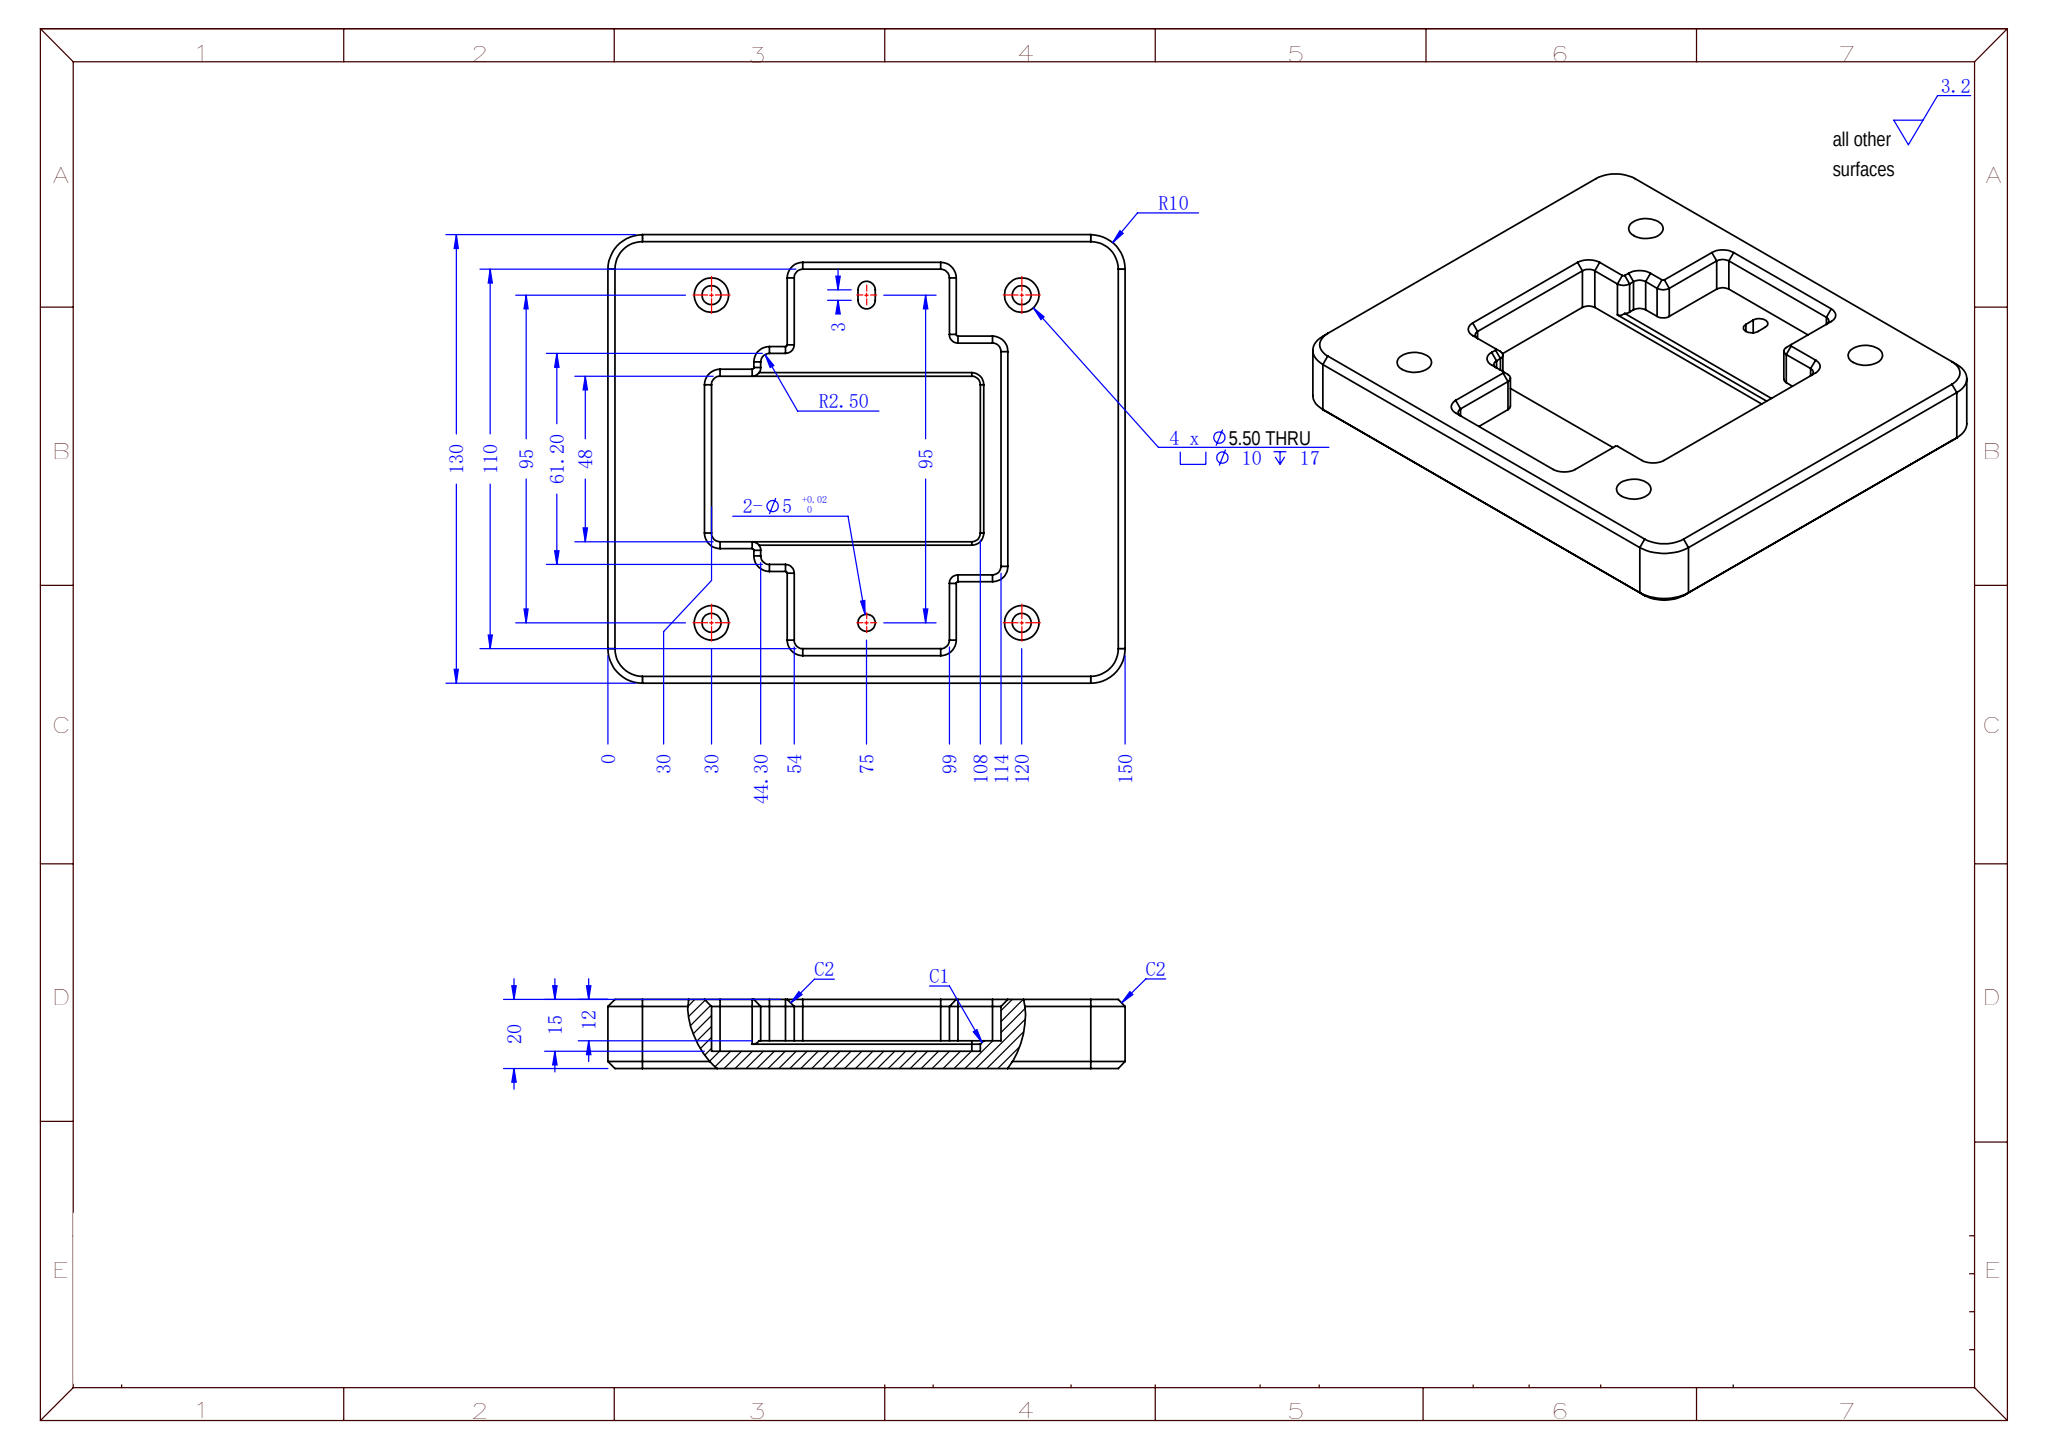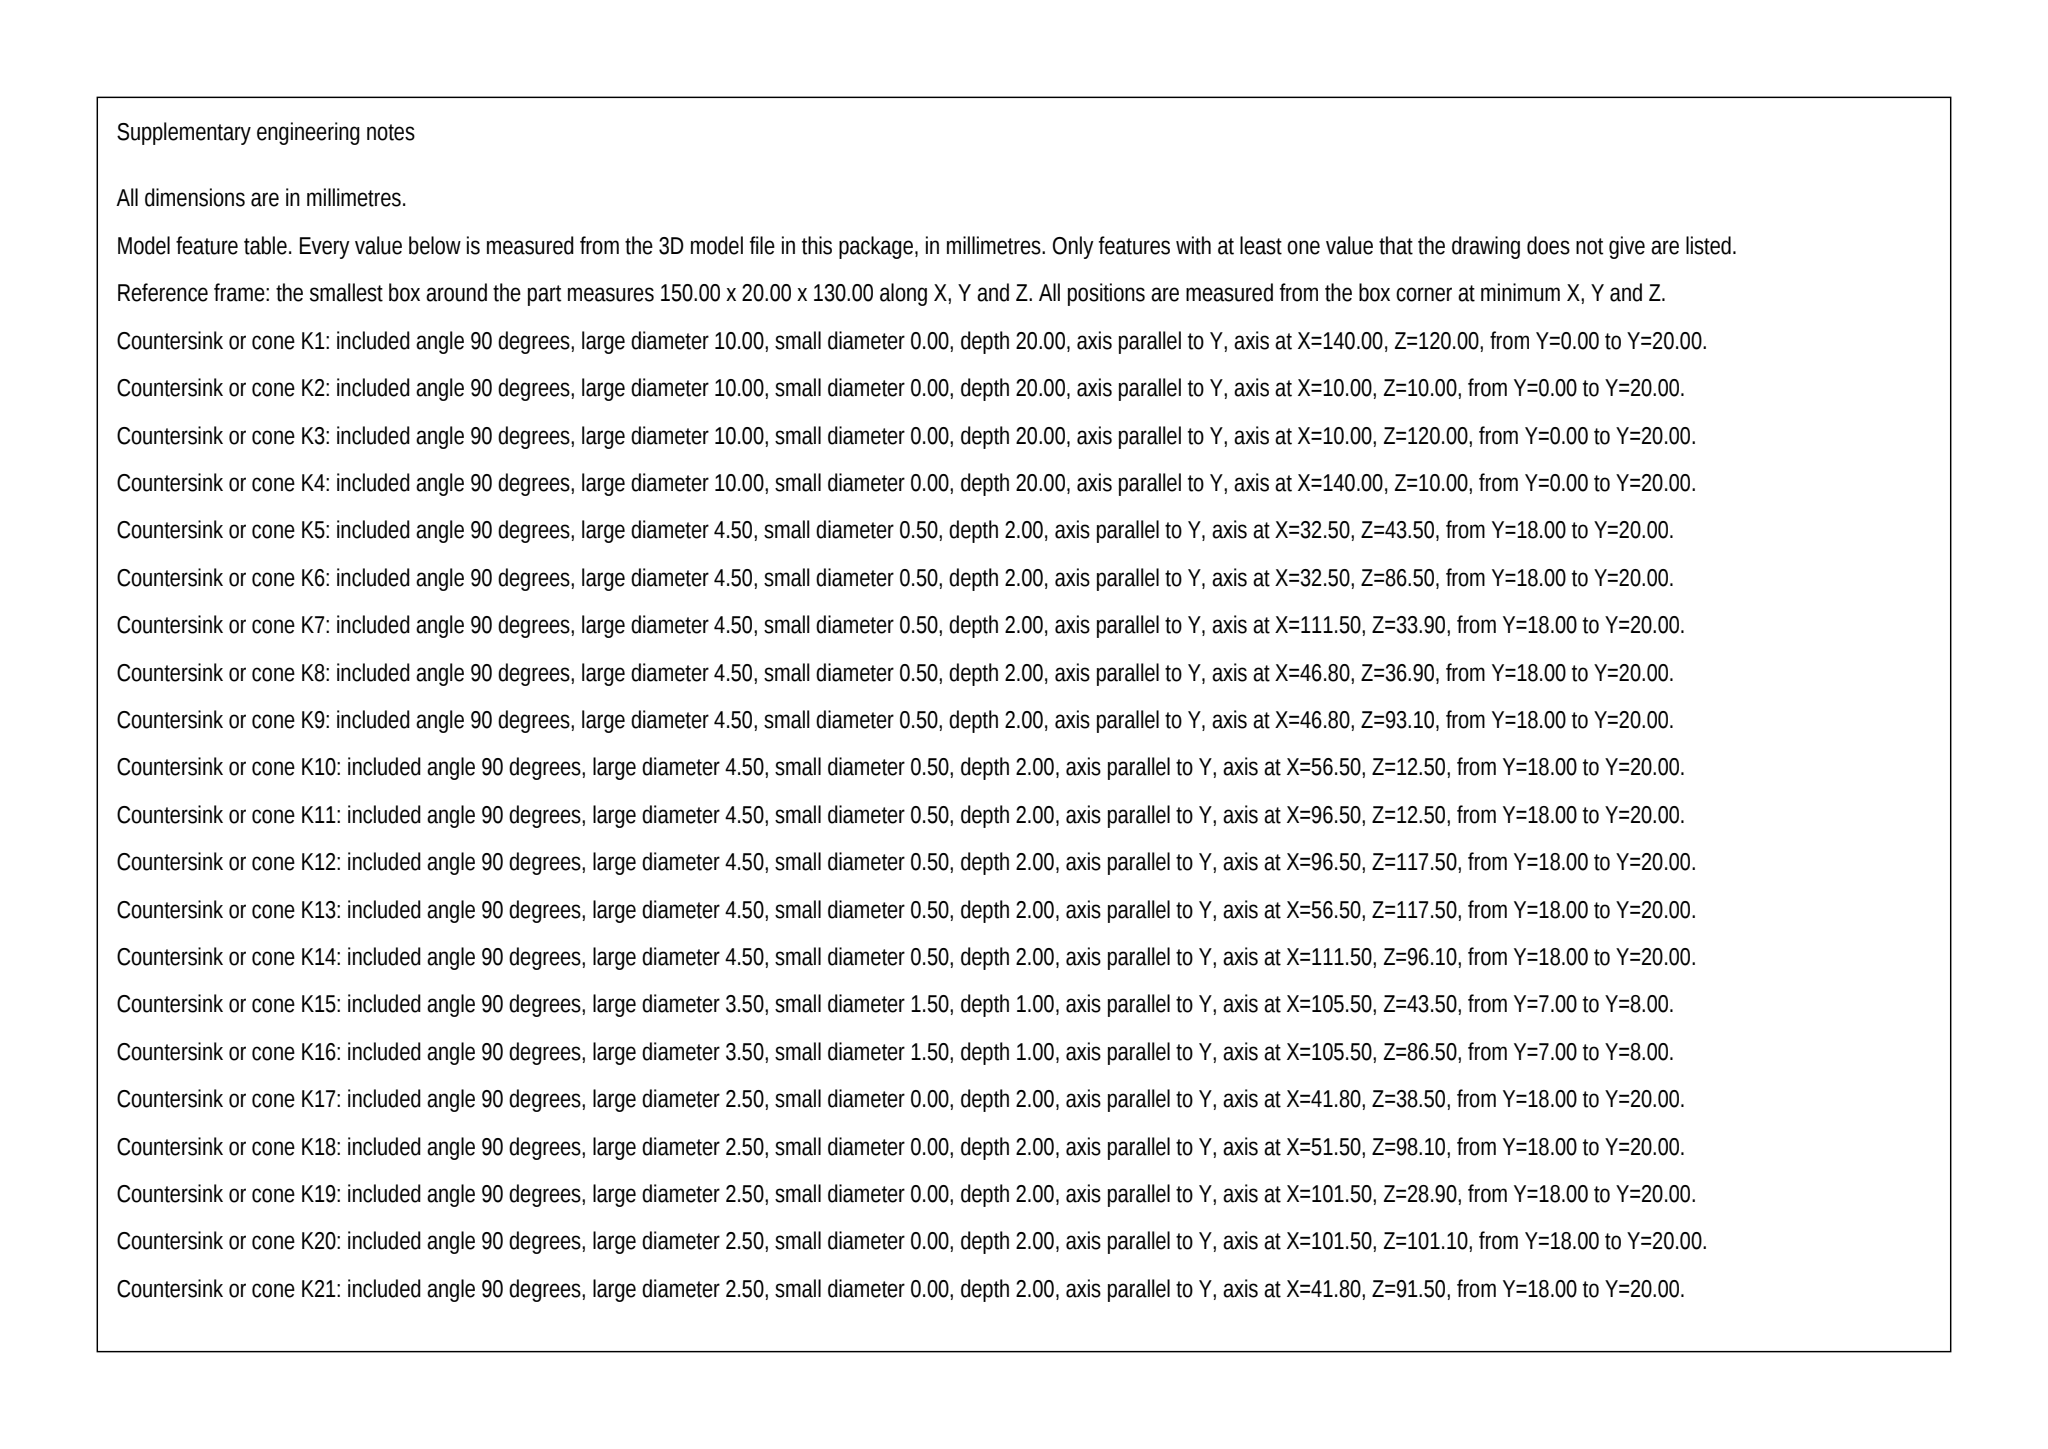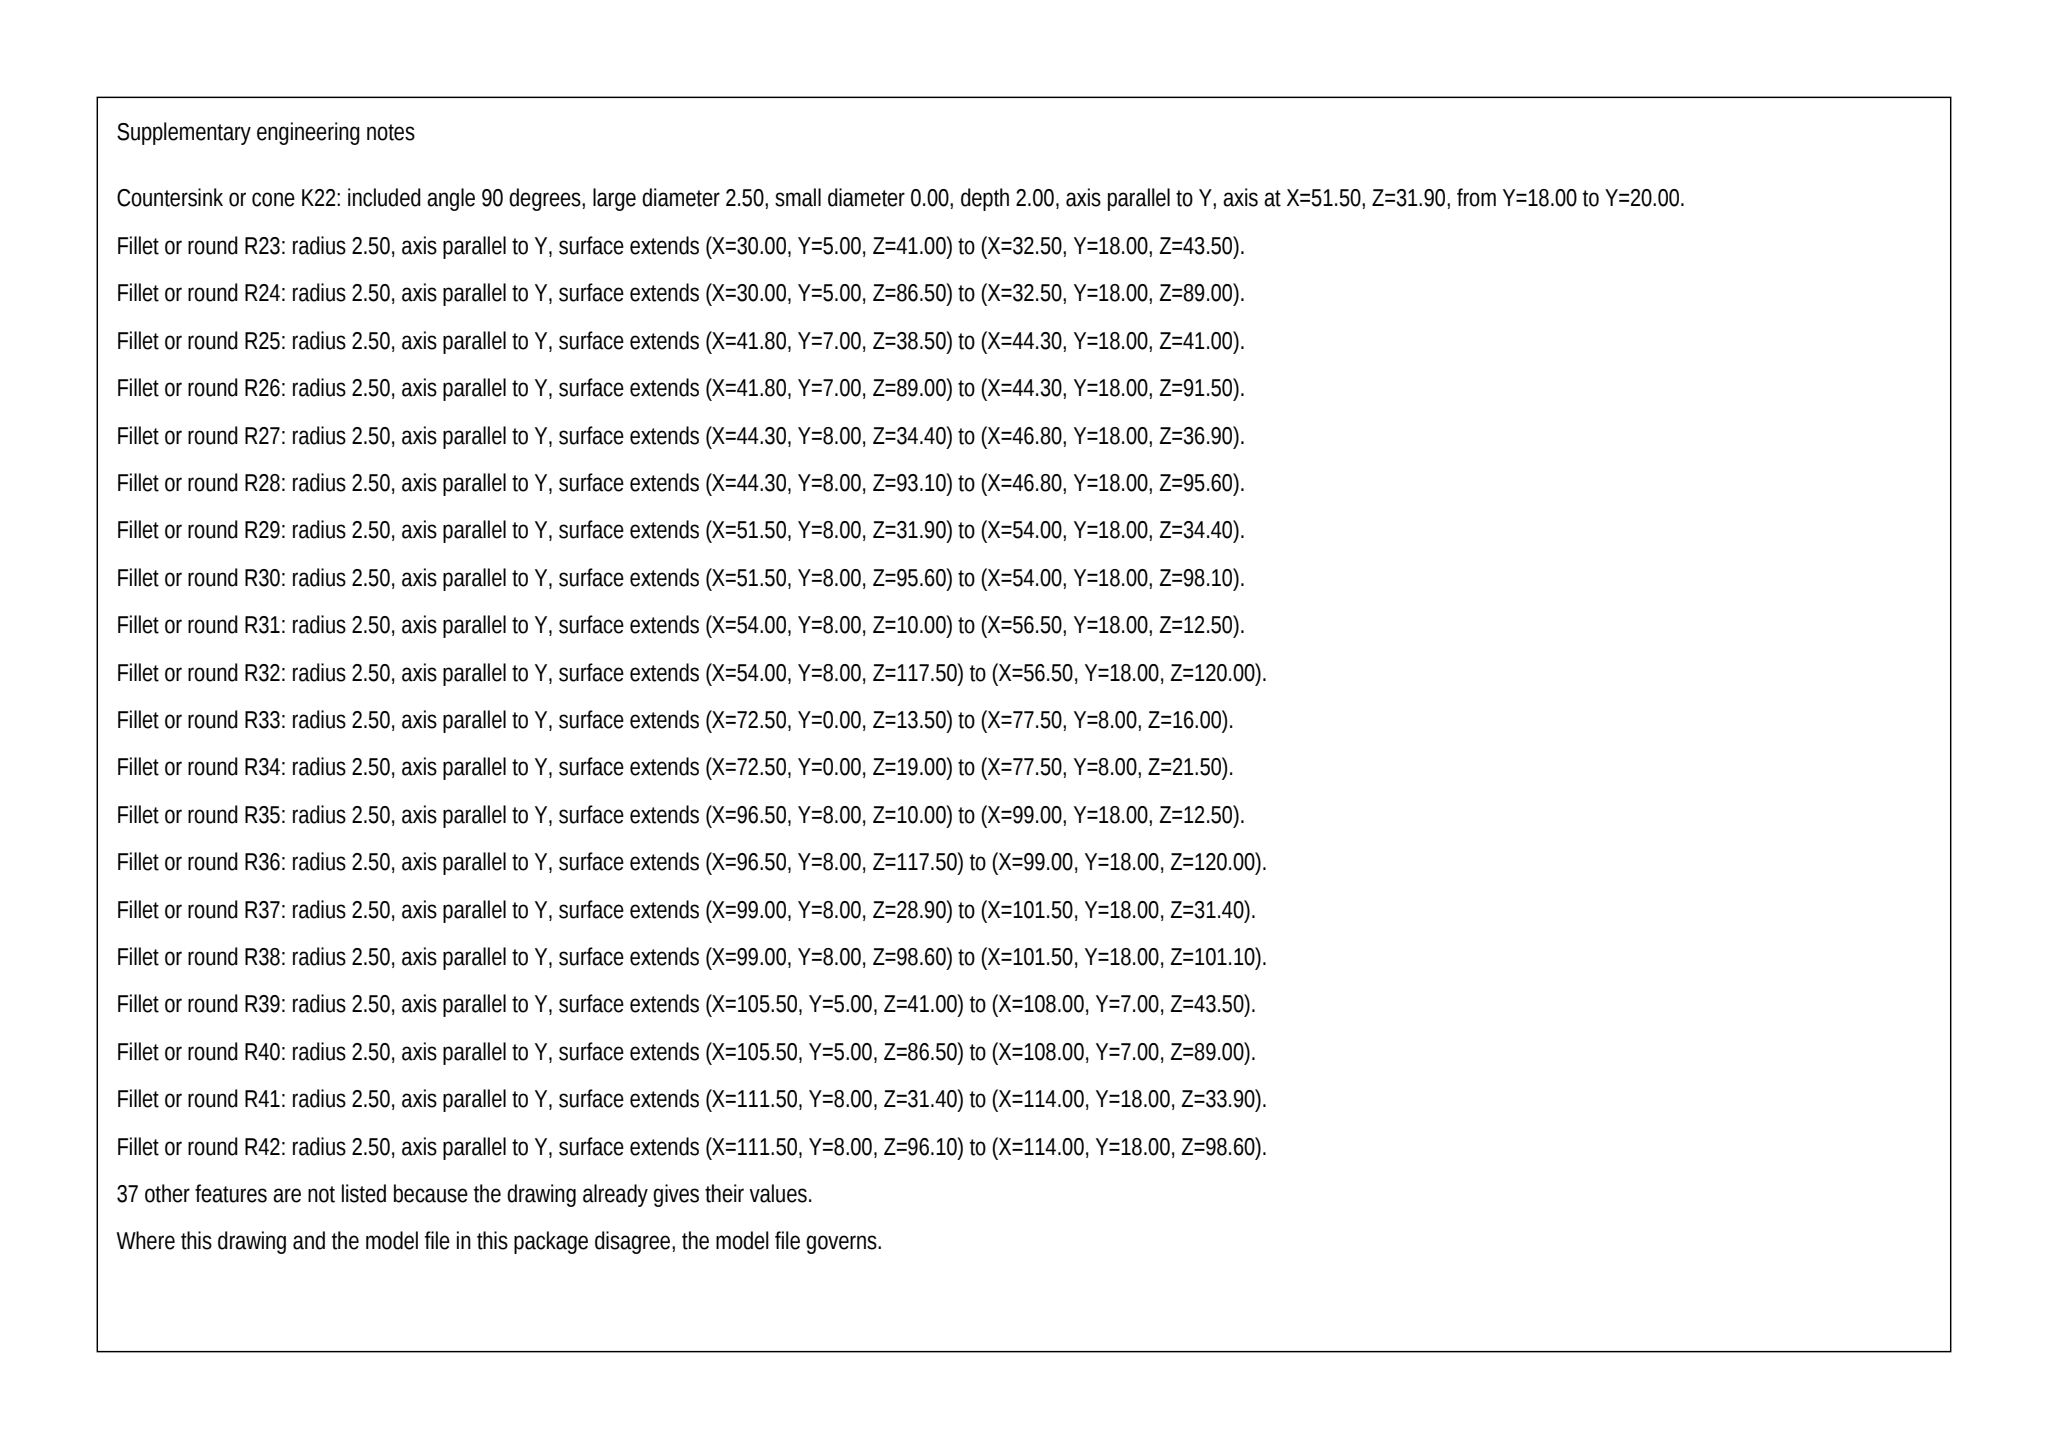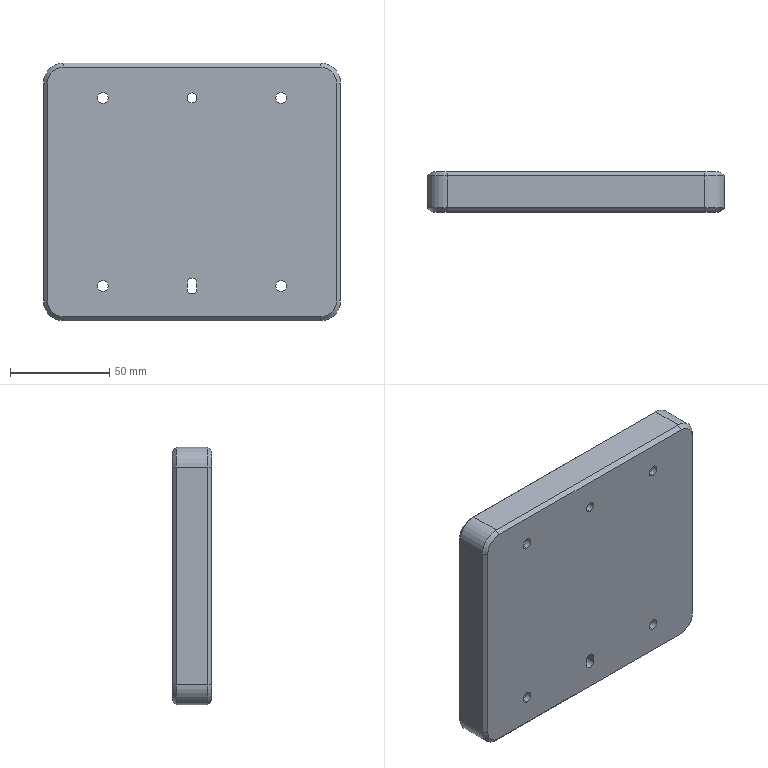Part | SolidWorks | mm | 1 solid | 127 faces | box 150 x 20 x 130 mm | volume 281222 mm3 | plane 58 | cylinder 43 | cone 26 | commonest cylinder face diameters 5 x23 10 x8 5.5 x8 20 x4
build123d program:
from build123d import *

# Parameters (mm, degrees)
SKETCH1_W                                       = 150
SKETCH1_H                                       = 130
BOSS_EXTRUDE1_DEPTH                             = 20
CUT_EXTRUDE2_DEPTH                              = 12
SKETCH2_W                                       = 78
SKETCH2_H                                       = 48
CUT_EXTRUDE1_DEPTH                              = 3
M5_HEX_SOCKET_HEAD_CAP_SCREW_CBORE1_D           = 5.5
M5_HEX_SOCKET_HEAD_CAP_SCREW_CBORE1_CBORE_D     = 10
M5_HEX_SOCKET_HEAD_CAP_SCREW_CBORE1_CBORE_DEPTH = 17
FILLET2_R                                       = 2.5
CHAMFER2_SIZE                                   = 1
CHAMFER3_SIZE                                   = 2
FILLET3_R                                       = 10
CHAMFER4_SIZE                                   = 2
CUT_EXTRUDE3_REACH                              = 101.97
SKETCH6_R                                       = 2.5


with BuildPart() as part:
    # Sketch1 → Boss-Extrude1 (new body)
    with BuildSketch(Plane(origin=(0, 0, 0), x_dir=(1, 0, 0), z_dir=(0, 1, 0))):
        Rectangle(SKETCH1_W, SKETCH1_H)
    extrude(amount=BOSS_EXTRUDE1_DEPTH)

    # Sketch3 → Cut-Extrude2 (cut)
    with BuildSketch(Plane(origin=(0, 20, 0), x_dir=(1, 0, 0), z_dir=(0, 1, 0))):
        Polygon((24, -33.6), (39, -33.6), (39, 33.6), (24, 33.6), (24, 55), (-21, 55), (-21, 30.6), (-30.7, 30.6), (-30.7, 24), (-45, 24), (-45, -24), (-30.7, -24), (-30.7, -30.6), (-21, -30.6), (-21, -55), (24, -55), align=None)
    extrude(amount=-CUT_EXTRUDE2_DEPTH, mode=Mode.SUBTRACT)

    # Sketch2 → Cut-Extrude1 (cut)
    with BuildSketch(Plane(origin=(0, 8, 0), x_dir=(1, 0, 0), z_dir=(0, 1, 0))):
        with Locations((-6, 0)):
            Rectangle(SKETCH2_W, SKETCH2_H)
    extrude(amount=-CUT_EXTRUDE1_DEPTH, mode=Mode.SUBTRACT)

    # M5 Hex Socket Head Cap Screw CBORE1 (through all)
    with Locations(Plane(origin=(0, 20, 0), x_dir=(1, 0, 0), z_dir=(0, 1, 0))):
        with Locations((-45, 47.5), (45, 47.5), (-45, -47.5), (45, -47.5)):
            CounterBoreHole(M5_HEX_SOCKET_HEAD_CAP_SCREW_CBORE1_D / 2, M5_HEX_SOCKET_HEAD_CAP_SCREW_CBORE1_CBORE_D / 2, M5_HEX_SOCKET_HEAD_CAP_SCREW_CBORE1_CBORE_DEPTH)

    # Fillet2
    fillet2_edges = [part.edges().sort_by_distance(p)[0] for p in [
        (24, 14, 33.6),
        (24, 14, 55),
        (-21, 14, 55),
        (-21, 14, 30.6),
        (-30.7, 14, 30.6),
        (-30.7, 14, 24),
        (-45, 12.5, 24),
        (-45, 12.5, -24),
        (-30.7, 14, -24),
        (-30.7, 14, -30.6),
        (-21, 14, -30.6),
        (-21, 14, -55),
        (24, 14, -55),
        (24, 14, -33.6),
        (39, 14, -33.6),
        (39, 14, 33.6),
        (33, 6.5, -24),
        (33, 6.5, 24),
    ]]
    fillet(fillet2_edges, radius=FILLET2_R)

    # Chamfer2
    chamfer2_edges = [part.edges().sort_by_distance(p)[0] for p in [
        (-1.35, 8, -24),
        (33, 8, 0),
        (32.268, 8, 23.268),
        (32.268, 8, -23.268),
        (-1.35, 8, 24),
    ]]
    chamfer(chamfer2_edges, length=CHAMFER2_SIZE)

    # Chamfer3
    chamfer3_edges = [part.edges().sort_by_distance(p)[0] for p in [
        (24, 20, -44.3),
        (24, 20, 44.3),
        (1.5, 20, 55),
        (-21, 20, 42.8),
        (-25.85, 20, 30.6),
        (-30.7, 20, 27.3),
        (-37.85, 20, 24),
        (-45, 20, 0),
        (-37.85, 20, -24),
        (-30.7, 20, -27.3),
        (-25.85, 20, -30.6),
        (-21, 20, -42.8),
        (1.5, 20, -55),
        (31.5, 20, -33.6),
        (39, 20, 0),
        (31.5, 20, 33.6),
        (24.732, 20, 34.332),
        (-21.732, 20, 31.332),
        (-31.432, 20, 24.732),
        (-31.432, 20, -24.732),
        (-21.732, 20, -31.332),
        (24.732, 20, -34.332),
        (-20.268, 20, -54.268),
        (23.268, 20, -54.268),
        (-44.268, 20, 23.268),
        (-44.268, 20, -23.268),
        (-29.968, 20, 29.868),
        (-20.268, 20, 54.268),
        (23.268, 20, 54.268),
        (38.268, 20, 32.868),
        (38.268, 20, -32.868),
        (-29.968, 20, -29.868),
    ]]
    chamfer(chamfer3_edges, length=CHAMFER3_SIZE)

    # Fillet3
    fillet3_edges = [part.edges().sort_by_distance(p)[0] for p in [
        (75, 10, 65),
        (-75, 10, 65),
        (-75, 10, -65),
        (75, 10, -65),
    ]]
    fillet(fillet3_edges, radius=FILLET3_R)

    # Chamfer4
    chamfer4_edges = [part.edges().sort_by_distance(p)[0] for p in [
        (75, 0, 0),
        (75, 20, 0),
        (0, 0, 65),
        (-75, 0, 0),
        (0, 0, -65),
        (-72.071, 0, 62.071),
        (72.071, 0, -62.071),
        (-72.071, 0, -62.071),
        (72.071, 0, 62.071),
        (0, 20, 65),
        (0, 20, -65),
        (-75, 20, 0),
        (-72.071, 20, 62.071),
        (72.071, 20, -62.071),
        (-72.071, 20, -62.071),
        (72.071, 20, 62.071),
    ]]
    chamfer(chamfer4_edges, length=CHAMFER4_SIZE)

    # Sketch6 → Cut-Extrude3 (cut, up to next)
    with BuildSketch(Plane(origin=(0, 8, 0), x_dir=(1, 0, 0), z_dir=(0, 1, 0)), mode=Mode.PRIVATE) as cut_extrude3_sk1:
        with Locations(Location((0, -47.5, 0), (0, 0, 270))):
            Circle(SKETCH6_R)
    cut_extrude3_tool1 = extrude(cut_extrude3_sk1.sketch, amount=-CUT_EXTRUDE3_REACH, mode=Mode.PRIVATE) & part.part
    # Sketch6 → Cut-Extrude3 (cut, up to next)
    with BuildSketch(Plane(origin=(0, 8, 0), x_dir=(1, 0, 0), z_dir=(0, 1, 0)), mode=Mode.PRIVATE) as cut_extrude3_sk2:
        with BuildLine():
            Line((2.5, 49), (2.5, 46))
            ThreePointArc((2.5, 46), (0, 43.5), (-2.5, 46))
            Line((-2.5, 46), (-2.5, 49))
            ThreePointArc((-2.5, 49), (0, 51.5), (2.5, 49))
        make_face()
    cut_extrude3_tool2 = extrude(cut_extrude3_sk2.sketch, amount=-CUT_EXTRUDE3_REACH, mode=Mode.PRIVATE) & part.part
    add(cut_extrude3_tool1.solids().sort_by_distance((0, 8, 47.5))[0], mode=Mode.SUBTRACT)
    add(cut_extrude3_tool2.solids().sort_by_distance((0, 8, -47.5))[0], mode=Mode.SUBTRACT)


solid = part.part